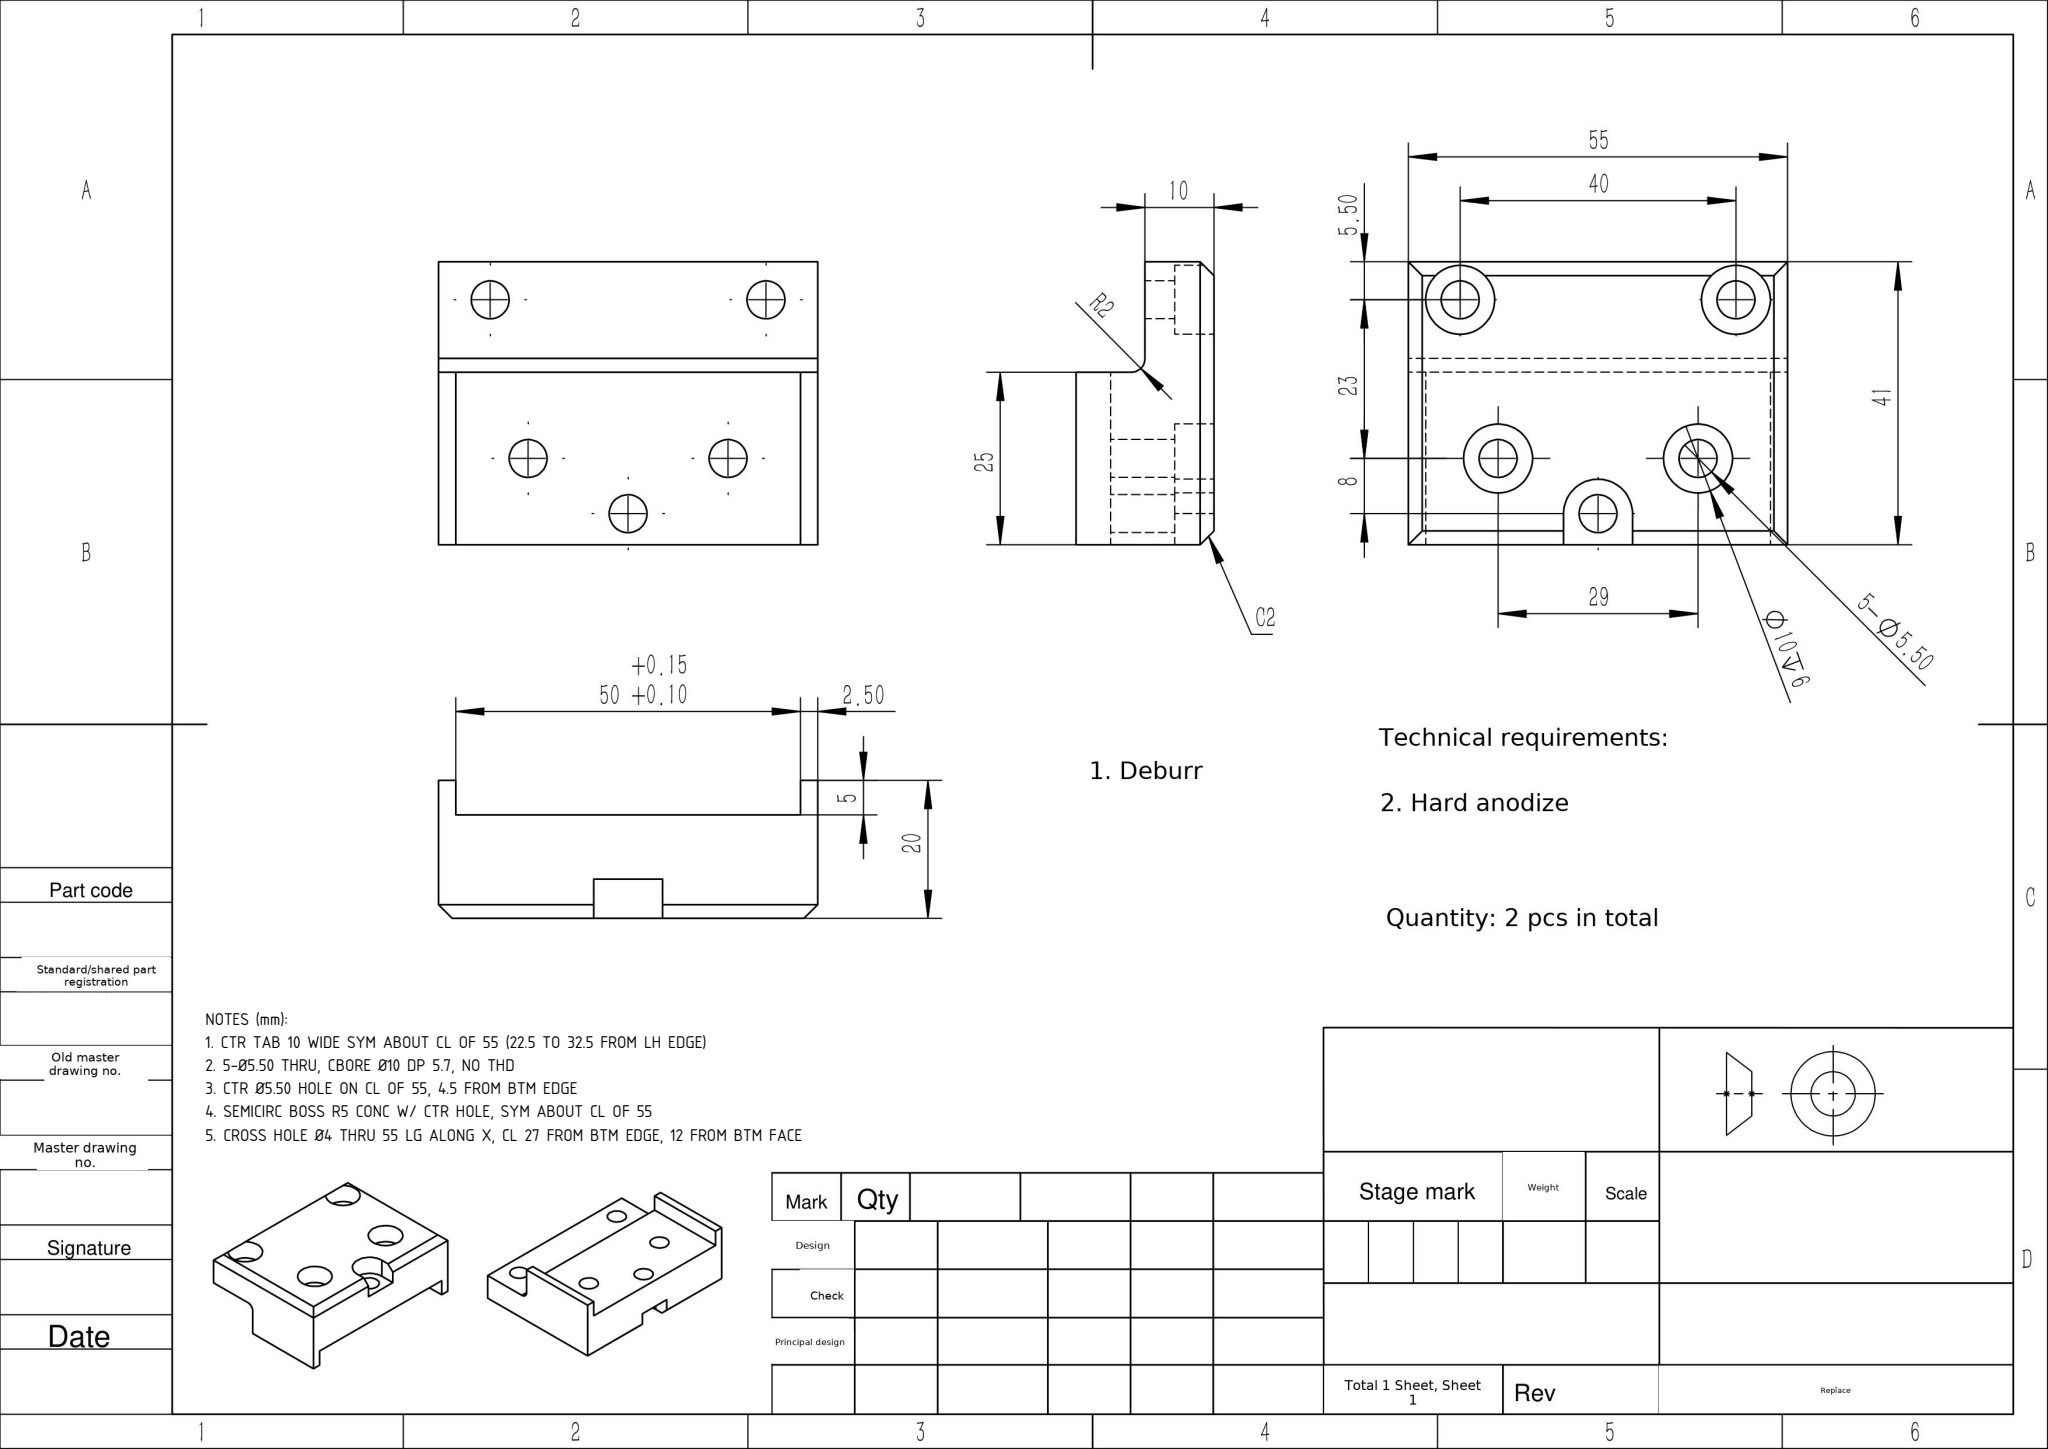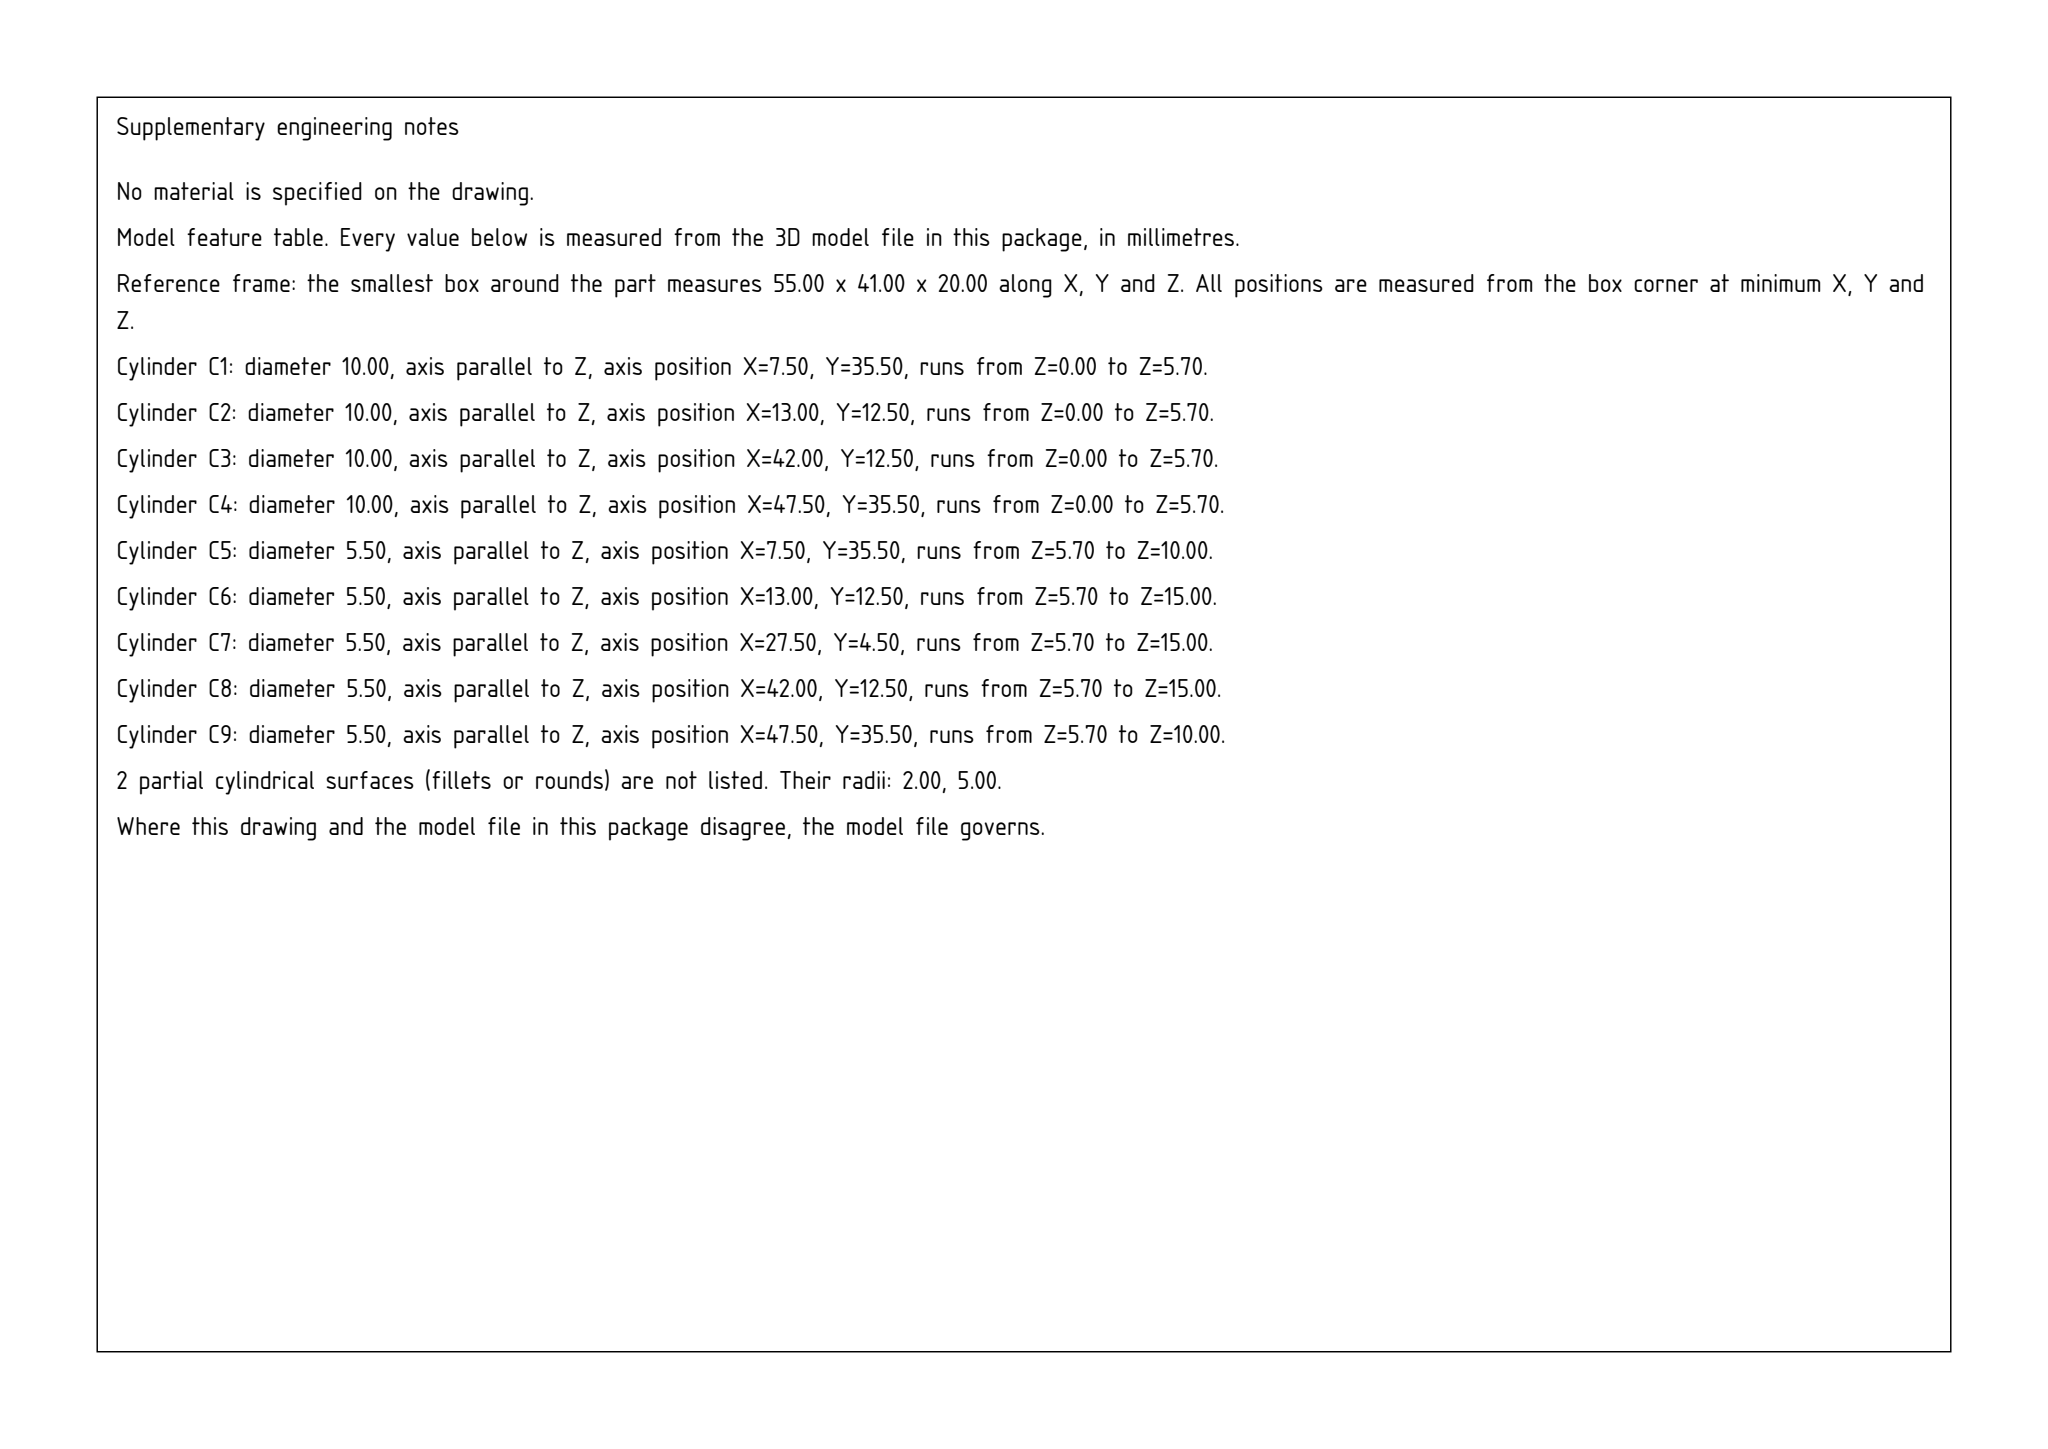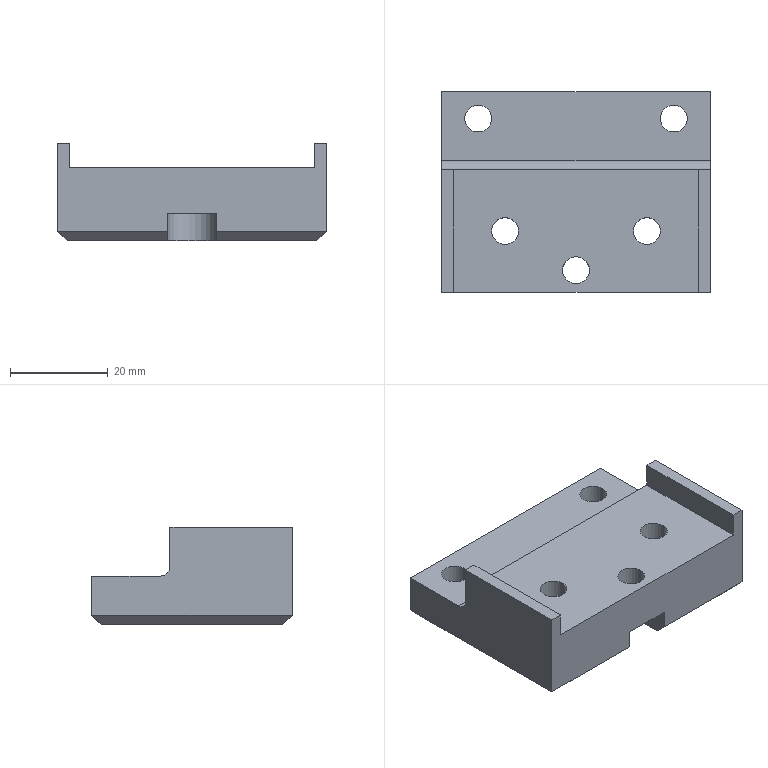Part | SolidWorks | mm | 1 solid | 44 faces | box 55 x 41 x 20 mm | volume 26615 mm3 | plane 24 | cylinder 20 | commonest cylinder face diameters 5.5 x10 10 x9 4 x1
Drawing notes:
CTR TAB 10 WIDE SYM ABOUT CL OF 55 (22.5 TO 32.5 FROM LH EDGE) | from the solid: x planes at 22.5 and 32.5 -> 10 wide, centered on 27.5 of 55
5-Ø5.50 THRU, CBORE Ø10 DP 5.7, NO THD | from the solid: 5x Ø5.5 z-cyls thru (4.3/9.3 to z=10/15) + 5x Ø10 cbore len 5.7, plane z=5.7
CTR Ø5.50 HOLE ON CL OF 55, 4.5 FROM BTM EDGE | from the solid: Ø5.5 & Ø10 z-cyls at (27.5,4.5); 27.5 = 55/2
SEMICIRC BOSS R5 CONC W/ CTR HOLE, SYM ABOUT CL OF 55 | from the solid: Ø10 cyl (count 1) at (27.5,4.5) at bottom edge, bbox y min 0
CROSS HOLE Ø4 THRU 55 LG ALONG X, CL 27 FROM BTM EDGE, 12 FROM BTM FACE | from the solid: cylinder dia 4.0, axis x, length 55.0, pos [null,27.0,12.0] from bbox min corner